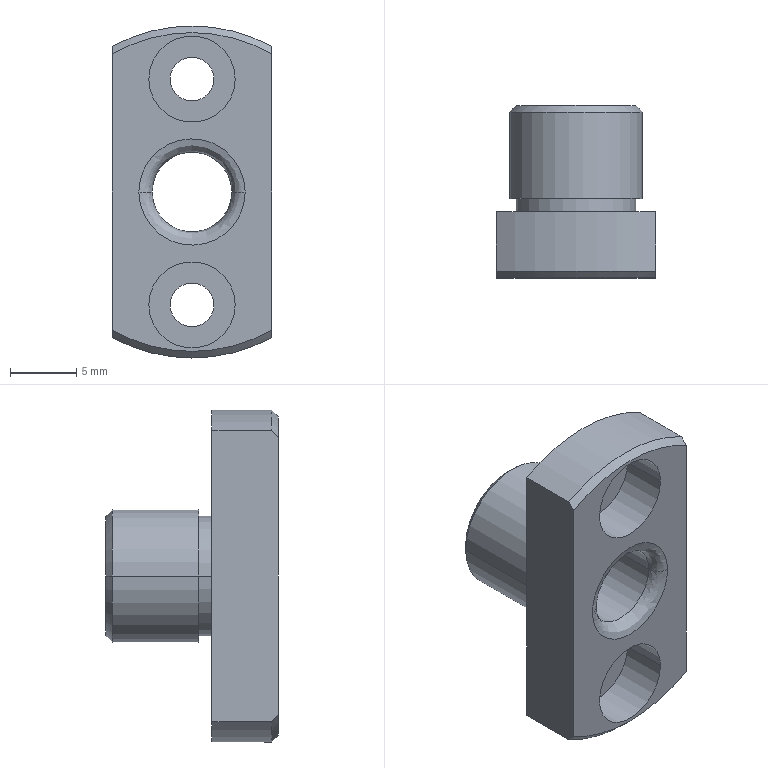Component | SolidWorks | F-JBNF10-P6-L8-1 | 1 solid | 30 faces | box 12 x 13 x 25 mm | volume 1417 mm3 | cylinder 16 | plane 8 | cone 4 | spline 2 | commonest cylinder face diameters 6.5 x4 3.3 x4 6 x2 10 x2 9 x2 25 x2
STEP:
#1=COLOUR_RGB('',0.7922,0.8196,0.9333);
#2=FILL_AREA_STYLE_COLOUR('',#1);
#3=FILL_AREA_STYLE('',(#2));
#4=SURFACE_STYLE_FILL_AREA(#3);
#5=SURFACE_SIDE_STYLE('',(#4));
#6=SURFACE_STYLE_USAGE(.BOTH.,#5);
#7=PRESENTATION_STYLE_ASSIGNMENT((#6));
#8=CARTESIAN_POINT('',(0.8391,-1.313,4.871));
#9=VERTEX_POINT('',#8);
#10=CARTESIAN_POINT('',(0.5241,-1.313,4.871));
#11=VERTEX_POINT('',#10);
#12=CARTESIAN_POINT('',(0.8391,-1.313,4.871));
#13=CARTESIAN_POINT('',(0.8391,-1.313,5.186));
#14=CARTESIAN_POINT('',(0.5241,-1.313,5.186));
#15=CARTESIAN_POINT('',(0.5241,-1.313,4.871));
#16=(BOUNDED_CURVE()B_SPLINE_CURVE(3,(#12,#13,#14,#15),.UNSPECIFIED.,.F.,.F.)B_SPLINE_CURVE_WITH_KNOTS((4,4),(0.,0.5),.UNSPECIFIED.)CURVE()GEOMETRIC_REPRESENTATION_ITEM()RATIONAL_B_SPLINE_CURVE((1.,0.3333,0.3333,1.))REPRESENTATION_ITEM(''));
#17=EDGE_CURVE('',#9,#11,#16,.T.);
#18=ORIENTED_EDGE('',*,*,#17,.T.);
#19=CARTESIAN_POINT('',(0.5635,-1.273,4.871));
#20=VERTEX_POINT('',#19);
#21=CARTESIAN_POINT('',(0.5241,-1.273,4.871));
#22=DIRECTION('',(-0.,0.,1.));
#23=DIRECTION('',(-1.,0.,0.));
#24=AXIS2_PLACEMENT_3D('',#21,#22,#23);
#25=CIRCLE('',#24,0.03937);
#26=EDGE_CURVE('',#11,#20,#25,.T.);
#27=ORIENTED_EDGE('',*,*,#26,.T.);
#28=CARTESIAN_POINT('',(0.7997,-1.273,4.871));
#29=VERTEX_POINT('',#28);
#30=CARTESIAN_POINT('',(0.6816,-1.273,4.871));
#31=DIRECTION('',(0.,1.,0.));
#32=DIRECTION('',(-1.,0.,0.));
#33=AXIS2_PLACEMENT_3D('',#30,#31,#32);
#34=CIRCLE('',#33,0.1181);
#35=EDGE_CURVE('',#20,#29,#34,.T.);
#36=ORIENTED_EDGE('',*,*,#35,.T.);
#37=CARTESIAN_POINT('',(0.8391,-1.273,4.871));
#38=DIRECTION('',(0.,0.,-1.));
#39=DIRECTION('',(1.,0.,0.));
#40=AXIS2_PLACEMENT_3D('',#37,#38,#39);
#41=CIRCLE('',#40,0.03937);
#42=EDGE_CURVE('',#9,#29,#41,.T.);
#43=ORIENTED_EDGE('',*,*,#42,.F.);
#44=EDGE_LOOP('',(#18,#27,#36,#43));
#45=FACE_OUTER_BOUND('',#44,.T.);
#46=CARTESIAN_POINT('',(0.5241,-1.313,4.871));
#47=CARTESIAN_POINT('',(0.5241,-1.313,5.186));
#48=CARTESIAN_POINT('',(0.8391,-1.313,5.186));
#49=CARTESIAN_POINT('',(0.8391,-1.313,4.871));
#50=CARTESIAN_POINT('',(0.5472,-1.313,4.871));
#51=CARTESIAN_POINT('',(0.5472,-1.313,5.14));
#52=CARTESIAN_POINT('',(0.816,-1.313,5.14));
#53=CARTESIAN_POINT('',(0.816,-1.313,4.871));
#54=CARTESIAN_POINT('',(0.5635,-1.296,4.871));
#55=CARTESIAN_POINT('',(0.5635,-1.296,5.107));
#56=CARTESIAN_POINT('',(0.7997,-1.296,5.107));
#57=CARTESIAN_POINT('',(0.7997,-1.296,4.871));
#58=CARTESIAN_POINT('',(0.5635,-1.273,4.871));
#59=CARTESIAN_POINT('',(0.5635,-1.273,5.107));
#60=CARTESIAN_POINT('',(0.7997,-1.273,5.107));
#61=CARTESIAN_POINT('',(0.7997,-1.273,4.871));
#62=(BOUNDED_SURFACE()B_SPLINE_SURFACE(3,3,((#46,#47,#48,#49),(#50,#51,#52,#53),(#54,#55,#56,#57),(#58,#59,#60,#61)),.UNSPECIFIED.,.F.,.F.,.F.)B_SPLINE_SURFACE_WITH_KNOTS((4,4),(4,4),(0.,1.),(0.,1.),.UNSPECIFIED.)GEOMETRIC_REPRESENTATION_ITEM()RATIONAL_B_SPLINE_SURFACE(((1.,0.3333,0.3333,1.),(0.8047,0.2682,0.2682,0.8047),(0.8047,0.2682,0.2682,0.8047),(1.,0.3333,0.3333,1.)))REPRESENTATION_ITEM('')SURFACE());
#63=ADVANCED_FACE('',(#45),#62,.T.);
#64=CARTESIAN_POINT('',(0.7997,-0.8009,4.871));
#65=VERTEX_POINT('',#64);
#66=CARTESIAN_POINT('',(0.5635,-0.8009,4.871));
#67=VERTEX_POINT('',#66);
#68=CARTESIAN_POINT('',(0.6816,-0.8009,4.871));
#69=DIRECTION('',(0.,-1.,0.));
#70=DIRECTION('',(-1.,0.,0.));
#71=AXIS2_PLACEMENT_3D('',#68,#69,#70);
#72=CIRCLE('',#71,0.1181);
#73=EDGE_CURVE('',#65,#67,#72,.T.);
#74=ORIENTED_EDGE('',*,*,#73,.F.);
#75=CARTESIAN_POINT('',(0.7997,-0.8009,4.871));
#76=DIRECTION('',(0.,-1.,0.));
#77=VECTOR('',#76,39.37);
#78=LINE('',#75,#77);
#79=EDGE_CURVE('',#65,#29,#78,.T.);
#80=ORIENTED_EDGE('',*,*,#79,.T.);
#81=ORIENTED_EDGE('',*,*,#35,.F.);
#82=CARTESIAN_POINT('',(0.5635,-0.8009,4.871));
#83=DIRECTION('',(0.,-1.,0.));
#84=VECTOR('',#83,39.37);
#85=LINE('',#82,#84);
#86=EDGE_CURVE('',#67,#20,#85,.T.);
#87=ORIENTED_EDGE('',*,*,#86,.F.);
#88=EDGE_LOOP('',(#74,#80,#81,#87));
#89=FACE_OUTER_BOUND('',#88,.T.);
#90=CARTESIAN_POINT('',(0.6816,-0.8009,4.871));
#91=DIRECTION('',(0.,-1.,0.));
#92=DIRECTION('',(-1.,0.,0.));
#93=AXIS2_PLACEMENT_3D('',#90,#91,#92);
#94=CYLINDRICAL_SURFACE('',#93,0.1181);
#95=ADVANCED_FACE('',(#89),#94,.F.);
#96=CARTESIAN_POINT('',(0.8587,-0.8009,4.871));
#97=VERTEX_POINT('',#96);
#98=CARTESIAN_POINT('',(0.5044,-0.8009,4.871));
#99=VERTEX_POINT('',#98);
#100=CARTESIAN_POINT('',(0.6816,-0.8009,4.871));
#101=DIRECTION('',(0.,1.,0.));
#102=DIRECTION('',(-1.,0.,0.));
#103=AXIS2_PLACEMENT_3D('',#100,#101,#102);
#104=CIRCLE('',#103,0.1772);
#105=EDGE_CURVE('',#97,#99,#104,.T.);
#106=ORIENTED_EDGE('',*,*,#105,.F.);
#107=CARTESIAN_POINT('',(0.8784,-0.8206,4.871));
#108=VERTEX_POINT('',#107);
#109=CARTESIAN_POINT('',(0.8784,-0.8206,4.871));
#110=DIRECTION('',(0.7071,-0.7071,-0.));
#111=VECTOR('',#110,39.37);
#112=LINE('',#109,#111);
#113=EDGE_CURVE('',#97,#108,#112,.T.);
#114=ORIENTED_EDGE('',*,*,#113,.T.);
#115=CARTESIAN_POINT('',(0.4847,-0.8206,4.871));
#116=VERTEX_POINT('',#115);
#117=CARTESIAN_POINT('',(0.6816,-0.8206,4.871));
#118=DIRECTION('',(0.,1.,0.));
#119=DIRECTION('',(-1.,0.,0.));
#120=AXIS2_PLACEMENT_3D('',#117,#118,#119);
#121=CIRCLE('',#120,0.1969);
#122=EDGE_CURVE('',#108,#116,#121,.T.);
#123=ORIENTED_EDGE('',*,*,#122,.T.);
#124=CARTESIAN_POINT('',(0.4847,-0.8206,4.871));
#125=DIRECTION('',(-0.7071,-0.7071,0.));
#126=VECTOR('',#125,39.37);
#127=LINE('',#124,#126);
#128=EDGE_CURVE('',#99,#116,#127,.T.);
#129=ORIENTED_EDGE('',*,*,#128,.F.);
#130=EDGE_LOOP('',(#106,#114,#123,#129));
#131=FACE_OUTER_BOUND('',#130,.T.);
#132=CARTESIAN_POINT('',(0.6816,-0.8206,4.871));
#133=DIRECTION('',(0.,-1.,0.));
#134=DIRECTION('',(-1.,0.,0.));
#135=AXIS2_PLACEMENT_3D('',#132,#133,#134);
#136=CONICAL_SURFACE('',#135,0.1969,0.7854);
#137=ADVANCED_FACE('',(#131),#136,.T.);
#138=CARTESIAN_POINT('',(0.5536,-1.313,5.206));
#139=VERTEX_POINT('',#138);
#140=CARTESIAN_POINT('',(0.8095,-1.313,5.206));
#141=VERTEX_POINT('',#140);
#142=CARTESIAN_POINT('',(0.6816,-1.313,5.206));
#143=DIRECTION('',(0.,1.,0.));
#144=DIRECTION('',(1.,0.,0.));
#145=AXIS2_PLACEMENT_3D('',#142,#143,#144);
#146=CIRCLE('',#145,0.128);
#147=EDGE_CURVE('',#139,#141,#146,.T.);
#148=ORIENTED_EDGE('',*,*,#147,.F.);
#149=CARTESIAN_POINT('',(0.5536,-1.175,5.206));
#150=VERTEX_POINT('',#149);
#151=CARTESIAN_POINT('',(0.5536,-1.313,5.206));
#152=DIRECTION('',(0.,1.,0.));
#153=VECTOR('',#152,39.37);
#154=LINE('',#151,#153);
#155=EDGE_CURVE('',#139,#150,#154,.T.);
#156=ORIENTED_EDGE('',*,*,#155,.T.);
#157=CARTESIAN_POINT('',(0.8095,-1.175,5.206));
#158=VERTEX_POINT('',#157);
#159=CARTESIAN_POINT('',(0.6816,-1.175,5.206));
#160=DIRECTION('',(0.,-1.,0.));
#161=DIRECTION('',(1.,0.,0.));
#162=AXIS2_PLACEMENT_3D('',#159,#160,#161);
#163=CIRCLE('',#162,0.128);
#164=EDGE_CURVE('',#158,#150,#163,.T.);
#165=ORIENTED_EDGE('',*,*,#164,.F.);
#166=CARTESIAN_POINT('',(0.8095,-1.313,5.206));
#167=DIRECTION('',(0.,1.,0.));
#168=VECTOR('',#167,39.37);
#169=LINE('',#166,#168);
#170=EDGE_CURVE('',#141,#158,#169,.T.);
#171=ORIENTED_EDGE('',*,*,#170,.F.);
#172=EDGE_LOOP('',(#148,#156,#165,#171));
#173=FACE_OUTER_BOUND('',#172,.T.);
#174=CARTESIAN_POINT('',(0.6816,-1.313,5.206));
#175=DIRECTION('',(0.,1.,0.));
#176=DIRECTION('',(1.,0.,0.));
#177=AXIS2_PLACEMENT_3D('',#174,#175,#176);
#178=CYLINDRICAL_SURFACE('',#177,0.128);
#179=ADVANCED_FACE('',(#173),#178,.F.);
#180=CARTESIAN_POINT('',(0.8095,-1.175,4.536));
#181=VERTEX_POINT('',#180);
#182=CARTESIAN_POINT('',(0.5536,-1.175,4.536));
#183=VERTEX_POINT('',#182);
#184=CARTESIAN_POINT('',(0.6816,-1.175,4.536));
#185=DIRECTION('',(0.,-1.,0.));
#186=DIRECTION('',(-1.,0.,0.));
#187=AXIS2_PLACEMENT_3D('',#184,#185,#186);
#188=CIRCLE('',#187,0.128);
#189=EDGE_CURVE('',#181,#183,#188,.T.);
#190=ORIENTED_EDGE('',*,*,#189,.F.);
#191=CARTESIAN_POINT('',(0.8095,-1.313,4.536));
#192=VERTEX_POINT('',#191);
#193=CARTESIAN_POINT('',(0.8095,-1.116,4.536));
#194=DIRECTION('',(0.,-1.,0.));
#195=VECTOR('',#194,39.37);
#196=LINE('',#193,#195);
#197=EDGE_CURVE('',#181,#192,#196,.T.);
#198=ORIENTED_EDGE('',*,*,#197,.T.);
#199=CARTESIAN_POINT('',(0.5536,-1.313,4.536));
#200=VERTEX_POINT('',#199);
#201=CARTESIAN_POINT('',(0.6816,-1.313,4.536));
#202=DIRECTION('',(0.,1.,0.));
#203=DIRECTION('',(-1.,0.,0.));
#204=AXIS2_PLACEMENT_3D('',#201,#202,#203);
#205=CIRCLE('',#204,0.128);
#206=EDGE_CURVE('',#200,#192,#205,.T.);
#207=ORIENTED_EDGE('',*,*,#206,.F.);
#208=CARTESIAN_POINT('',(0.5536,-1.116,4.536));
#209=DIRECTION('',(0.,-1.,0.));
#210=VECTOR('',#209,39.37);
#211=LINE('',#208,#210);
#212=EDGE_CURVE('',#183,#200,#211,.T.);
#213=ORIENTED_EDGE('',*,*,#212,.F.);
#214=EDGE_LOOP('',(#190,#198,#207,#213));
#215=FACE_OUTER_BOUND('',#214,.T.);
#216=CARTESIAN_POINT('',(0.6816,-1.116,4.536));
#217=DIRECTION('',(0.,-1.,0.));
#218=DIRECTION('',(-1.,0.,0.));
#219=AXIS2_PLACEMENT_3D('',#216,#217,#218);
#220=CYLINDRICAL_SURFACE('',#219,0.128);
#221=ADVANCED_FACE('',(#215),#220,.F.);
#222=ORIENTED_EDGE('',*,*,#122,.F.);
#223=CARTESIAN_POINT('',(0.8784,-1.076,4.871));
#224=VERTEX_POINT('',#223);
#225=CARTESIAN_POINT('',(0.8784,-0.8009,4.871));
#226=DIRECTION('',(0.,-1.,0.));
#227=VECTOR('',#226,39.37);
#228=LINE('',#225,#227);
#229=EDGE_CURVE('',#108,#224,#228,.T.);
#230=ORIENTED_EDGE('',*,*,#229,.T.);
#231=CARTESIAN_POINT('',(0.4847,-1.076,4.871));
#232=VERTEX_POINT('',#231);
#233=CARTESIAN_POINT('',(0.6816,-1.076,4.871));
#234=DIRECTION('',(0.,1.,0.));
#235=DIRECTION('',(-1.,0.,0.));
#236=AXIS2_PLACEMENT_3D('',#233,#234,#235);
#237=CIRCLE('',#236,0.1969);
#238=EDGE_CURVE('',#224,#232,#237,.T.);
#239=ORIENTED_EDGE('',*,*,#238,.T.);
#240=CARTESIAN_POINT('',(0.4847,-0.8009,4.871));
#241=DIRECTION('',(0.,-1.,0.));
#242=VECTOR('',#241,39.37);
#243=LINE('',#240,#242);
#244=EDGE_CURVE('',#116,#232,#243,.T.);
#245=ORIENTED_EDGE('',*,*,#244,.F.);
#246=EDGE_LOOP('',(#222,#230,#239,#245));
#247=FACE_OUTER_BOUND('',#246,.T.);
#248=CARTESIAN_POINT('',(0.6816,-0.8009,4.871));
#249=DIRECTION('',(0.,-1.,0.));
#250=DIRECTION('',(-1.,0.,0.));
#251=AXIS2_PLACEMENT_3D('',#248,#249,#250);
#252=CYLINDRICAL_SURFACE('',#251,0.1969);
#253=ADVANCED_FACE('',(#247),#252,.T.);
#254=CARTESIAN_POINT('',(0.6166,-1.175,5.206));
#255=VERTEX_POINT('',#254);
#256=CARTESIAN_POINT('',(0.7465,-1.175,5.206));
#257=VERTEX_POINT('',#256);
#258=CARTESIAN_POINT('',(0.6816,-1.175,5.206));
#259=DIRECTION('',(0.,1.,0.));
#260=DIRECTION('',(1.,0.,0.));
#261=AXIS2_PLACEMENT_3D('',#258,#259,#260);
#262=CIRCLE('',#261,0.06496);
#263=EDGE_CURVE('',#255,#257,#262,.T.);
#264=ORIENTED_EDGE('',*,*,#263,.F.);
#265=CARTESIAN_POINT('',(0.6166,-1.116,5.206));
#266=VERTEX_POINT('',#265);
#267=CARTESIAN_POINT('',(0.6166,-1.313,5.206));
#268=DIRECTION('',(0.,1.,0.));
#269=VECTOR('',#268,39.37);
#270=LINE('',#267,#269);
#271=EDGE_CURVE('',#255,#266,#270,.T.);
#272=ORIENTED_EDGE('',*,*,#271,.T.);
#273=CARTESIAN_POINT('',(0.7465,-1.116,5.206));
#274=VERTEX_POINT('',#273);
#275=CARTESIAN_POINT('',(0.6816,-1.116,5.206));
#276=DIRECTION('',(0.,-1.,0.));
#277=DIRECTION('',(1.,0.,0.));
#278=AXIS2_PLACEMENT_3D('',#275,#276,#277);
#279=CIRCLE('',#278,0.06496);
#280=EDGE_CURVE('',#274,#266,#279,.T.);
#281=ORIENTED_EDGE('',*,*,#280,.F.);
#282=CARTESIAN_POINT('',(0.7465,-1.313,5.206));
#283=DIRECTION('',(0.,1.,0.));
#284=VECTOR('',#283,39.37);
#285=LINE('',#282,#284);
#286=EDGE_CURVE('',#257,#274,#285,.T.);
#287=ORIENTED_EDGE('',*,*,#286,.F.);
#288=EDGE_LOOP('',(#264,#272,#281,#287));
#289=FACE_OUTER_BOUND('',#288,.T.);
#290=CARTESIAN_POINT('',(0.6816,-1.313,5.206));
#291=DIRECTION('',(0.,1.,0.));
#292=DIRECTION('',(1.,0.,0.));
#293=AXIS2_PLACEMENT_3D('',#290,#291,#292);
#294=CYLINDRICAL_SURFACE('',#293,0.06496);
#295=ADVANCED_FACE('',(#289),#294,.F.);
#296=CARTESIAN_POINT('',(0.8587,-1.076,4.871));
#297=VERTEX_POINT('',#296);
#298=CARTESIAN_POINT('',(0.5044,-1.076,4.871));
#299=VERTEX_POINT('',#298);
#300=CARTESIAN_POINT('',(0.6816,-1.076,4.871));
#301=DIRECTION('',(0.,1.,0.));
#302=DIRECTION('',(-1.,0.,0.));
#303=AXIS2_PLACEMENT_3D('',#300,#301,#302);
#304=CIRCLE('',#303,0.1772);
#305=EDGE_CURVE('',#297,#299,#304,.T.);
#306=ORIENTED_EDGE('',*,*,#305,.F.);
#307=CARTESIAN_POINT('',(0.8587,-1.116,4.871));
#308=VERTEX_POINT('',#307);
#309=CARTESIAN_POINT('',(0.8587,-0.8009,4.871));
#310=DIRECTION('',(0.,-1.,0.));
#311=VECTOR('',#310,39.37);
#312=LINE('',#309,#311);
#313=EDGE_CURVE('',#297,#308,#312,.T.);
#314=ORIENTED_EDGE('',*,*,#313,.T.);
#315=CARTESIAN_POINT('',(0.5044,-1.116,4.871));
#316=VERTEX_POINT('',#315);
#317=CARTESIAN_POINT('',(0.6816,-1.116,4.871));
#318=DIRECTION('',(0.,-1.,0.));
#319=DIRECTION('',(-1.,0.,0.));
#320=AXIS2_PLACEMENT_3D('',#317,#318,#319);
#321=CIRCLE('',#320,0.1772);
#322=EDGE_CURVE('',#316,#308,#321,.T.);
#323=ORIENTED_EDGE('',*,*,#322,.F.);
#324=CARTESIAN_POINT('',(0.5044,-0.8009,4.871));
#325=DIRECTION('',(0.,-1.,0.));
#326=VECTOR('',#325,39.37);
#327=LINE('',#324,#326);
#328=EDGE_CURVE('',#299,#316,#327,.T.);
#329=ORIENTED_EDGE('',*,*,#328,.F.);
#330=EDGE_LOOP('',(#306,#314,#323,#329));
#331=FACE_OUTER_BOUND('',#330,.T.);
#332=CARTESIAN_POINT('',(0.6816,-0.8009,4.871));
#333=DIRECTION('',(0.,-1.,0.));
#334=DIRECTION('',(-1.,0.,0.));
#335=AXIS2_PLACEMENT_3D('',#332,#333,#334);
#336=CYLINDRICAL_SURFACE('',#335,0.1772);
#337=ADVANCED_FACE('',(#331),#336,.T.);
#338=CARTESIAN_POINT('',(0.7465,-1.116,4.536));
#339=VERTEX_POINT('',#338);
#340=CARTESIAN_POINT('',(0.6166,-1.116,4.536));
#341=VERTEX_POINT('',#340);
#342=CARTESIAN_POINT('',(0.6816,-1.116,4.536));
#343=DIRECTION('',(0.,-1.,0.));
#344=DIRECTION('',(-1.,0.,0.));
#345=AXIS2_PLACEMENT_3D('',#342,#343,#344);
#346=CIRCLE('',#345,0.06496);
#347=EDGE_CURVE('',#339,#341,#346,.T.);
#348=ORIENTED_EDGE('',*,*,#347,.F.);
#349=CARTESIAN_POINT('',(0.7465,-1.175,4.536));
#350=VERTEX_POINT('',#349);
#351=CARTESIAN_POINT('',(0.7465,-1.116,4.536));
#352=DIRECTION('',(0.,-1.,0.));
#353=VECTOR('',#352,39.37);
#354=LINE('',#351,#353);
#355=EDGE_CURVE('',#339,#350,#354,.T.);
#356=ORIENTED_EDGE('',*,*,#355,.T.);
#357=CARTESIAN_POINT('',(0.6166,-1.175,4.536));
#358=VERTEX_POINT('',#357);
#359=CARTESIAN_POINT('',(0.6816,-1.175,4.536));
#360=DIRECTION('',(0.,1.,0.));
#361=DIRECTION('',(-1.,0.,0.));
#362=AXIS2_PLACEMENT_3D('',#359,#360,#361);
#363=CIRCLE('',#362,0.06496);
#364=EDGE_CURVE('',#358,#350,#363,.T.);
#365=ORIENTED_EDGE('',*,*,#364,.F.);
#366=CARTESIAN_POINT('',(0.6166,-1.116,4.536));
#367=DIRECTION('',(0.,-1.,0.));
#368=VECTOR('',#367,39.37);
#369=LINE('',#366,#368);
#370=EDGE_CURVE('',#341,#358,#369,.T.);
#371=ORIENTED_EDGE('',*,*,#370,.F.);
#372=EDGE_LOOP('',(#348,#356,#365,#371));
#373=FACE_OUTER_BOUND('',#372,.T.);
#374=CARTESIAN_POINT('',(0.6816,-1.116,4.536));
#375=DIRECTION('',(0.,-1.,0.));
#376=DIRECTION('',(-1.,0.,0.));
#377=AXIS2_PLACEMENT_3D('',#374,#375,#376);
#378=CYLINDRICAL_SURFACE('',#377,0.06496);
#379=ADVANCED_FACE('',(#373),#378,.F.);
#380=ORIENTED_EDGE('',*,*,#79,.F.);
#381=CARTESIAN_POINT('',(0.6816,-0.8009,4.871));
#382=DIRECTION('',(0.,-1.,0.));
#383=DIRECTION('',(-1.,0.,0.));
#384=AXIS2_PLACEMENT_3D('',#381,#382,#383);
#385=CIRCLE('',#384,0.1181);
#386=EDGE_CURVE('',#67,#65,#385,.T.);
#387=ORIENTED_EDGE('',*,*,#386,.F.);
#388=ORIENTED_EDGE('',*,*,#86,.T.);
#389=CARTESIAN_POINT('',(0.6816,-1.273,4.871));
#390=DIRECTION('',(0.,1.,0.));
#391=DIRECTION('',(-1.,0.,0.));
#392=AXIS2_PLACEMENT_3D('',#389,#390,#391);
#393=CIRCLE('',#392,0.1181);
#394=EDGE_CURVE('',#29,#20,#393,.T.);
#395=ORIENTED_EDGE('',*,*,#394,.F.);
#396=EDGE_LOOP('',(#380,#387,#388,#395));
#397=FACE_OUTER_BOUND('',#396,.T.);
#398=CARTESIAN_POINT('',(0.6816,-0.8009,4.871));
#399=DIRECTION('',(0.,-1.,0.));
#400=DIRECTION('',(-1.,0.,0.));
#401=AXIS2_PLACEMENT_3D('',#398,#399,#400);
#402=CYLINDRICAL_SURFACE('',#401,0.1181);
#403=ADVANCED_FACE('',(#397),#402,.F.);
#404=ORIENTED_EDGE('',*,*,#26,.F.);
#405=CARTESIAN_POINT('',(0.5241,-1.313,4.871));
#406=CARTESIAN_POINT('',(0.5241,-1.313,4.556));
#407=CARTESIAN_POINT('',(0.8391,-1.313,4.556));
#408=CARTESIAN_POINT('',(0.8391,-1.313,4.871));
#409=(BOUNDED_CURVE()B_SPLINE_CURVE(3,(#405,#406,#407,#408),.UNSPECIFIED.,.F.,.F.)B_SPLINE_CURVE_WITH_KNOTS((4,4),(0.5,1.),.UNSPECIFIED.)CURVE()GEOMETRIC_REPRESENTATION_ITEM()RATIONAL_B_SPLINE_CURVE((1.,0.3333,0.3333,1.))REPRESENTATION_ITEM(''));
#410=EDGE_CURVE('',#11,#9,#409,.T.);
#411=ORIENTED_EDGE('',*,*,#410,.T.);
#412=ORIENTED_EDGE('',*,*,#42,.T.);
#413=ORIENTED_EDGE('',*,*,#394,.T.);
#414=EDGE_LOOP('',(#404,#411,#412,#413));
#415=FACE_OUTER_BOUND('',#414,.T.);
#416=CARTESIAN_POINT('',(0.8391,-1.313,4.871));
#417=CARTESIAN_POINT('',(0.8391,-1.313,4.556));
#418=CARTESIAN_POINT('',(0.5241,-1.313,4.556));
#419=CARTESIAN_POINT('',(0.5241,-1.313,4.871));
#420=CARTESIAN_POINT('',(0.816,-1.313,4.871));
#421=CARTESIAN_POINT('',(0.816,-1.313,4.602));
#422=CARTESIAN_POINT('',(0.5472,-1.313,4.602));
#423=CARTESIAN_POINT('',(0.5472,-1.313,4.871));
#424=CARTESIAN_POINT('',(0.7997,-1.296,4.871));
#425=CARTESIAN_POINT('',(0.7997,-1.296,4.635));
#426=CARTESIAN_POINT('',(0.5635,-1.296,4.635));
#427=CARTESIAN_POINT('',(0.5635,-1.296,4.871));
#428=CARTESIAN_POINT('',(0.7997,-1.273,4.871));
#429=CARTESIAN_POINT('',(0.7997,-1.273,4.635));
#430=CARTESIAN_POINT('',(0.5635,-1.273,4.635));
#431=CARTESIAN_POINT('',(0.5635,-1.273,4.871));
#432=(BOUNDED_SURFACE()B_SPLINE_SURFACE(3,3,((#416,#417,#418,#419),(#420,#421,#422,#423),(#424,#425,#426,#427),(#428,#429,#430,#431)),.UNSPECIFIED.,.F.,.F.,.F.)B_SPLINE_SURFACE_WITH_KNOTS((4,4),(4,4),(0.,1.),(0.,1.),.UNSPECIFIED.)GEOMETRIC_REPRESENTATION_ITEM()RATIONAL_B_SPLINE_SURFACE(((1.,0.3333,0.3333,1.),(0.8047,0.2682,0.2682,0.8047),(0.8047,0.2682,0.2682,0.8047),(1.,0.3333,0.3333,1.)))REPRESENTATION_ITEM('')SURFACE());
#433=ADVANCED_FACE('',(#415),#432,.T.);
#434=ORIENTED_EDGE('',*,*,#386,.T.);
#435=ORIENTED_EDGE('',*,*,#73,.T.);
#436=EDGE_LOOP('',(#434,#435));
#437=FACE_BOUND('',#436,.T.);
#438=CARTESIAN_POINT('',(0.6816,-0.8009,4.871));
#439=DIRECTION('',(0.,1.,0.));
#440=DIRECTION('',(-1.,0.,0.));
#441=AXIS2_PLACEMENT_3D('',#438,#439,#440);
#442=CIRCLE('',#441,0.1772);
#443=EDGE_CURVE('',#99,#97,#442,.T.);
#444=ORIENTED_EDGE('',*,*,#443,.T.);
#445=ORIENTED_EDGE('',*,*,#105,.T.);
#446=EDGE_LOOP('',(#444,#445));
#447=FACE_OUTER_BOUND('',#446,.T.);
#448=CARTESIAN_POINT('',(0.6816,-0.8009,4.753));
#449=DIRECTION('',(0.,1.,0.));
#450=DIRECTION('',(1.,0.,0.));
#451=AXIS2_PLACEMENT_3D('',#448,#449,#450);
#452=PLANE('',#451);
#453=ADVANCED_FACE('',(#437,#447),#452,.T.);
#454=CARTESIAN_POINT('',(0.6816,-1.313,5.206));
#455=DIRECTION('',(0.,1.,0.));
#456=DIRECTION('',(1.,0.,0.));
#457=AXIS2_PLACEMENT_3D('',#454,#455,#456);
#458=CIRCLE('',#457,0.128);
#459=EDGE_CURVE('',#141,#139,#458,.T.);
#460=ORIENTED_EDGE('',*,*,#459,.T.);
#461=ORIENTED_EDGE('',*,*,#147,.T.);
#462=EDGE_LOOP('',(#460,#461));
#463=FACE_BOUND('',#462,.T.);
#464=CARTESIAN_POINT('',(0.9178,-1.313,5.28));
#465=VERTEX_POINT('',#464);
#466=CARTESIAN_POINT('',(0.4454,-1.313,5.28));
#467=VERTEX_POINT('',#466);
#468=CARTESIAN_POINT('',(0.6816,-1.313,4.871));
#469=DIRECTION('',(0.,-1.,0.));
#470=DIRECTION('',(1.,0.,-0.));
#471=AXIS2_PLACEMENT_3D('',#468,#469,#470);
#472=CIRCLE('',#471,0.4724);
#473=EDGE_CURVE('',#465,#467,#472,.T.);
#474=ORIENTED_EDGE('',*,*,#473,.T.);
#475=CARTESIAN_POINT('',(0.4454,-1.313,4.462));
#476=VERTEX_POINT('',#475);
#477=CARTESIAN_POINT('',(0.4454,-1.313,4.398));
#478=DIRECTION('',(0.,0.,-1.));
#479=VECTOR('',#478,39.37);
#480=LINE('',#477,#479);
#481=EDGE_CURVE('',#467,#476,#480,.T.);
#482=ORIENTED_EDGE('',*,*,#481,.T.);
#483=CARTESIAN_POINT('',(0.9178,-1.313,4.462));
#484=VERTEX_POINT('',#483);
#485=CARTESIAN_POINT('',(0.6816,-1.313,4.871));
#486=DIRECTION('',(0.,-1.,0.));
#487=DIRECTION('',(1.,0.,0.));
#488=AXIS2_PLACEMENT_3D('',#485,#486,#487);
#489=CIRCLE('',#488,0.4724);
#490=EDGE_CURVE('',#476,#484,#489,.T.);
#491=ORIENTED_EDGE('',*,*,#490,.T.);
#492=CARTESIAN_POINT('',(0.9178,-1.313,4.398));
#493=DIRECTION('',(0.,0.,1.));
#494=VECTOR('',#493,39.37);
#495=LINE('',#492,#494);
#496=EDGE_CURVE('',#484,#465,#495,.T.);
#497=ORIENTED_EDGE('',*,*,#496,.T.);
#498=EDGE_LOOP('',(#474,#482,#491,#497));
#499=FACE_OUTER_BOUND('',#498,.T.);
#500=ORIENTED_EDGE('',*,*,#206,.T.);
#501=CARTESIAN_POINT('',(0.6816,-1.313,4.536));
#502=DIRECTION('',(0.,1.,0.));
#503=DIRECTION('',(-1.,0.,0.));
#504=AXIS2_PLACEMENT_3D('',#501,#502,#503);
#505=CIRCLE('',#504,0.128);
#506=EDGE_CURVE('',#192,#200,#505,.T.);
#507=ORIENTED_EDGE('',*,*,#506,.T.);
#508=EDGE_LOOP('',(#500,#507));
#509=FACE_BOUND('',#508,.T.);
#510=ORIENTED_EDGE('',*,*,#17,.F.);
#511=ORIENTED_EDGE('',*,*,#410,.F.);
#512=EDGE_LOOP('',(#510,#511));
#513=FACE_BOUND('',#512,.T.);
#514=CARTESIAN_POINT('',(0.6816,-1.313,4.398));
#515=DIRECTION('',(0.,-1.,0.));
#516=DIRECTION('',(-1.,0.,0.));
#517=AXIS2_PLACEMENT_3D('',#514,#515,#516);
#518=PLANE('',#517);
#519=ADVANCED_FACE('',(#463,#499,#509,#513),#518,.T.);
#520=ORIENTED_EDGE('',*,*,#113,.F.);
#521=ORIENTED_EDGE('',*,*,#443,.F.);
#522=ORIENTED_EDGE('',*,*,#128,.T.);
#523=CARTESIAN_POINT('',(0.6816,-0.8206,4.871));
#524=DIRECTION('',(0.,1.,0.));
#525=DIRECTION('',(-1.,0.,0.));
#526=AXIS2_PLACEMENT_3D('',#523,#524,#525);
#527=CIRCLE('',#526,0.1969);
#528=EDGE_CURVE('',#116,#108,#527,.T.);
#529=ORIENTED_EDGE('',*,*,#528,.T.);
#530=EDGE_LOOP('',(#520,#521,#522,#529));
#531=FACE_OUTER_BOUND('',#530,.T.);
#532=CARTESIAN_POINT('',(0.6816,-0.8206,4.871));
#533=DIRECTION('',(0.,-1.,0.));
#534=DIRECTION('',(-1.,0.,0.));
#535=AXIS2_PLACEMENT_3D('',#532,#533,#534);
#536=CONICAL_SURFACE('',#535,0.1969,0.7854);
#537=ADVANCED_FACE('',(#531),#536,.T.);
#538=ORIENTED_EDGE('',*,*,#155,.F.);
#539=ORIENTED_EDGE('',*,*,#459,.F.);
#540=ORIENTED_EDGE('',*,*,#170,.T.);
#541=CARTESIAN_POINT('',(0.6816,-1.175,5.206));
#542=DIRECTION('',(0.,-1.,0.));
#543=DIRECTION('',(1.,0.,0.));
#544=AXIS2_PLACEMENT_3D('',#541,#542,#543);
#545=CIRCLE('',#544,0.128);
#546=EDGE_CURVE('',#150,#158,#545,.T.);
#547=ORIENTED_EDGE('',*,*,#546,.F.);
#548=EDGE_LOOP('',(#538,#539,#540,#547));
#549=FACE_OUTER_BOUND('',#548,.T.);
#550=CARTESIAN_POINT('',(0.6816,-1.313,5.206));
#551=DIRECTION('',(0.,1.,0.));
#552=DIRECTION('',(1.,0.,0.));
#553=AXIS2_PLACEMENT_3D('',#550,#551,#552);
#554=CYLINDRICAL_SURFACE('',#553,0.128);
#555=ADVANCED_FACE('',(#549),#554,.F.);
#556=CARTESIAN_POINT('',(0.4454,-1.293,4.439));
#557=VERTEX_POINT('',#556);
#558=CARTESIAN_POINT('',(0.4454,-1.313,4.462));
#559=CARTESIAN_POINT('',(0.4454,-1.306,4.454));
#560=CARTESIAN_POINT('',(0.4454,-1.3,4.447));
#561=CARTESIAN_POINT('',(0.4454,-1.293,4.439));
#562=B_SPLINE_CURVE_WITH_KNOTS('',3,(#558,#559,#560,#561),.UNSPECIFIED.,.F.,.F.,(4,4),(0.,0.0007609),.UNSPECIFIED.);
#563=EDGE_CURVE('',#476,#557,#562,.T.);
#564=ORIENTED_EDGE('',*,*,#563,.F.);
#565=ORIENTED_EDGE('',*,*,#481,.F.);
#566=CARTESIAN_POINT('',(0.4454,-1.293,5.303));
#567=VERTEX_POINT('',#566);
#568=CARTESIAN_POINT('',(0.4454,-1.293,5.303));
#569=CARTESIAN_POINT('',(0.4454,-1.3,5.295));
#570=CARTESIAN_POINT('',(0.4454,-1.306,5.288));
#571=CARTESIAN_POINT('',(0.4454,-1.313,5.28));
#572=B_SPLINE_CURVE_WITH_KNOTS('',3,(#568,#569,#570,#571),.UNSPECIFIED.,.F.,.F.,(4,4),(0.,0.0007609),.UNSPECIFIED.);
#573=EDGE_CURVE('',#567,#467,#572,.T.);
#574=ORIENTED_EDGE('',*,*,#573,.F.);
#575=CARTESIAN_POINT('',(0.4454,-1.116,5.303));
#576=VERTEX_POINT('',#575);
#577=CARTESIAN_POINT('',(0.4454,-1.116,5.303));
#578=DIRECTION('',(0.,-1.,0.));
#579=VECTOR('',#578,39.37);
#580=LINE('',#577,#579);
#581=EDGE_CURVE('',#576,#567,#580,.T.);
#582=ORIENTED_EDGE('',*,*,#581,.F.);
#583=CARTESIAN_POINT('',(0.4454,-1.116,4.439));
#584=VERTEX_POINT('',#583);
#585=CARTESIAN_POINT('',(0.4454,-1.116,4.379));
#586=DIRECTION('',(0.,0.,1.));
#587=VECTOR('',#586,39.37);
#588=LINE('',#585,#587);
#589=EDGE_CURVE('',#584,#576,#588,.T.);
#590=ORIENTED_EDGE('',*,*,#589,.F.);
#591=CARTESIAN_POINT('',(0.4454,-1.116,4.439));
#592=DIRECTION('',(0.,1.,0.));
#593=VECTOR('',#592,39.37);
#594=LINE('',#591,#593);
#595=EDGE_CURVE('',#557,#584,#594,.T.);
#596=ORIENTED_EDGE('',*,*,#595,.F.);
#597=EDGE_LOOP('',(#564,#565,#574,#582,#590,#596));
#598=FACE_OUTER_BOUND('',#597,.T.);
#599=CARTESIAN_POINT('',(0.4454,-1.116,4.379));
#600=DIRECTION('',(1.,0.,0.));
#601=DIRECTION('',(0.,-1.,0.));
#602=AXIS2_PLACEMENT_3D('',#599,#600,#601);
#603=PLANE('',#602);
#604=ADVANCED_FACE('',(#598),#603,.F.);
#605=CARTESIAN_POINT('',(0.9178,-1.293,5.303));
#606=VERTEX_POINT('',#605);
#607=CARTESIAN_POINT('',(0.9178,-1.313,5.28));
#608=CARTESIAN_POINT('',(0.9178,-1.306,5.288));
#609=CARTESIAN_POINT('',(0.9178,-1.3,5.295));
#610=CARTESIAN_POINT('',(0.9178,-1.293,5.303));
#611=B_SPLINE_CURVE_WITH_KNOTS('',3,(#607,#608,#609,#610),.UNSPECIFIED.,.F.,.F.,(4,4),(0.,0.0007609),.UNSPECIFIED.);
#612=EDGE_CURVE('',#465,#606,#611,.T.);
#613=ORIENTED_EDGE('',*,*,#612,.T.);
#614=CARTESIAN_POINT('',(0.6816,-1.293,4.871));
#615=DIRECTION('',(0.,-1.,0.));
#616=DIRECTION('',(1.,0.,-0.));
#617=AXIS2_PLACEMENT_3D('',#614,#615,#616);
#618=CIRCLE('',#617,0.4921);
#619=EDGE_CURVE('',#606,#567,#618,.T.);
#620=ORIENTED_EDGE('',*,*,#619,.T.);
#621=ORIENTED_EDGE('',*,*,#573,.T.);
#622=ORIENTED_EDGE('',*,*,#473,.F.);
#623=EDGE_LOOP('',(#613,#620,#621,#622));
#624=FACE_OUTER_BOUND('',#623,.T.);
#625=CARTESIAN_POINT('',(0.6816,-1.293,4.871));
#626=DIRECTION('',(0.,1.,0.));
#627=DIRECTION('',(1.,0.,0.));
#628=AXIS2_PLACEMENT_3D('',#625,#626,#627);
#629=CONICAL_SURFACE('',#628,0.4921,0.7854);
#630=ADVANCED_FACE('',(#624),#629,.T.);
#631=ORIENTED_EDGE('',*,*,#612,.F.);
#632=ORIENTED_EDGE('',*,*,#496,.F.);
#633=CARTESIAN_POINT('',(0.9178,-1.293,4.439));
#634=VERTEX_POINT('',#633);
#635=CARTESIAN_POINT('',(0.9178,-1.293,4.439));
#636=CARTESIAN_POINT('',(0.9178,-1.3,4.447));
#637=CARTESIAN_POINT('',(0.9178,-1.306,4.454));
#638=CARTESIAN_POINT('',(0.9178,-1.313,4.462));
#639=B_SPLINE_CURVE_WITH_KNOTS('',3,(#635,#636,#637,#638),.UNSPECIFIED.,.F.,.F.,(4,4),(0.,0.0007609),.UNSPECIFIED.);
#640=EDGE_CURVE('',#634,#484,#639,.T.);
#641=ORIENTED_EDGE('',*,*,#640,.F.);
#642=CARTESIAN_POINT('',(0.9178,-1.116,4.439));
#643=VERTEX_POINT('',#642);
#644=CARTESIAN_POINT('',(0.9178,-1.116,4.439));
#645=DIRECTION('',(0.,-1.,0.));
#646=VECTOR('',#645,39.37);
#647=LINE('',#644,#646);
#648=EDGE_CURVE('',#643,#634,#647,.T.);
#649=ORIENTED_EDGE('',*,*,#648,.F.);
#650=CARTESIAN_POINT('',(0.9178,-1.116,5.303));
#651=VERTEX_POINT('',#650);
#652=CARTESIAN_POINT('',(0.9178,-1.116,5.363));
#653=DIRECTION('',(0.,0.,-1.));
#654=VECTOR('',#653,39.37);
#655=LINE('',#652,#654);
#656=EDGE_CURVE('',#651,#643,#655,.T.);
#657=ORIENTED_EDGE('',*,*,#656,.F.);
#658=CARTESIAN_POINT('',(0.9178,-1.116,5.303));
#659=DIRECTION('',(0.,1.,0.));
#660=VECTOR('',#659,39.37);
#661=LINE('',#658,#660);
#662=EDGE_CURVE('',#606,#651,#661,.T.);
#663=ORIENTED_EDGE('',*,*,#662,.F.);
#664=EDGE_LOOP('',(#631,#632,#641,#649,#657,#663));
#665=FACE_OUTER_BOUND('',#664,.T.);
#666=CARTESIAN_POINT('',(0.9178,-1.116,5.363));
#667=DIRECTION('',(-1.,0.,0.));
#668=DIRECTION('',(0.,1.,0.));
#669=AXIS2_PLACEMENT_3D('',#666,#667,#668);
#670=PLANE('',#669);
#671=ADVANCED_FACE('',(#665),#670,.F.);
#672=ORIENTED_EDGE('',*,*,#563,.T.);
#673=CARTESIAN_POINT('',(0.6816,-1.293,4.871));
#674=DIRECTION('',(0.,-1.,0.));
#675=DIRECTION('',(1.,0.,0.));
#676=AXIS2_PLACEMENT_3D('',#673,#674,#675);
#677=CIRCLE('',#676,0.4921);
#678=EDGE_CURVE('',#557,#634,#677,.T.);
#679=ORIENTED_EDGE('',*,*,#678,.T.);
#680=ORIENTED_EDGE('',*,*,#640,.T.);
#681=ORIENTED_EDGE('',*,*,#490,.F.);
#682=EDGE_LOOP('',(#672,#679,#680,#681));
#683=FACE_OUTER_BOUND('',#682,.T.);
#684=CARTESIAN_POINT('',(0.6816,-1.293,4.871));
#685=DIRECTION('',(0.,1.,0.));
#686=DIRECTION('',(1.,0.,0.));
#687=AXIS2_PLACEMENT_3D('',#684,#685,#686);
#688=CONICAL_SURFACE('',#687,0.4921,0.7854);
#689=ADVANCED_FACE('',(#683),#688,.T.);
#690=ORIENTED_EDGE('',*,*,#197,.F.);
#691=CARTESIAN_POINT('',(0.6816,-1.175,4.536));
#692=DIRECTION('',(0.,-1.,0.));
#693=DIRECTION('',(-1.,0.,0.));
#694=AXIS2_PLACEMENT_3D('',#691,#692,#693);
#695=CIRCLE('',#694,0.128);
#696=EDGE_CURVE('',#183,#181,#695,.T.);
#697=ORIENTED_EDGE('',*,*,#696,.F.);
#698=ORIENTED_EDGE('',*,*,#212,.T.);
#699=ORIENTED_EDGE('',*,*,#506,.F.);
#700=EDGE_LOOP('',(#690,#697,#698,#699));
#701=FACE_OUTER_BOUND('',#700,.T.);
#702=CARTESIAN_POINT('',(0.6816,-1.116,4.536));
#703=DIRECTION('',(0.,-1.,0.));
#704=DIRECTION('',(-1.,0.,0.));
#705=AXIS2_PLACEMENT_3D('',#702,#703,#704);
#706=CYLINDRICAL_SURFACE('',#705,0.128);
#707=ADVANCED_FACE('',(#701),#706,.F.);
#708=ORIENTED_EDGE('',*,*,#229,.F.);
#709=ORIENTED_EDGE('',*,*,#528,.F.);
#710=ORIENTED_EDGE('',*,*,#244,.T.);
#711=CARTESIAN_POINT('',(0.6816,-1.076,4.871));
#712=DIRECTION('',(0.,1.,0.));
#713=DIRECTION('',(-1.,0.,0.));
#714=AXIS2_PLACEMENT_3D('',#711,#712,#713);
#715=CIRCLE('',#714,0.1969);
#716=EDGE_CURVE('',#232,#224,#715,.T.);
#717=ORIENTED_EDGE('',*,*,#716,.T.);
#718=EDGE_LOOP('',(#708,#709,#710,#717));
#719=FACE_OUTER_BOUND('',#718,.T.);
#720=CARTESIAN_POINT('',(0.6816,-0.8009,4.871));
#721=DIRECTION('',(0.,-1.,0.));
#722=DIRECTION('',(-1.,0.,0.));
#723=AXIS2_PLACEMENT_3D('',#720,#721,#722);
#724=CYLINDRICAL_SURFACE('',#723,0.1969);
#725=ADVANCED_FACE('',(#719),#724,.T.);
#726=CARTESIAN_POINT('',(0.6816,-1.175,5.206));
#727=DIRECTION('',(0.,1.,0.));
#728=DIRECTION('',(1.,0.,0.));
#729=AXIS2_PLACEMENT_3D('',#726,#727,#728);
#730=CIRCLE('',#729,0.06496);
#731=EDGE_CURVE('',#257,#255,#730,.T.);
#732=ORIENTED_EDGE('',*,*,#731,.T.);
#733=ORIENTED_EDGE('',*,*,#263,.T.);
#734=EDGE_LOOP('',(#732,#733));
#735=FACE_BOUND('',#734,.T.);
#736=ORIENTED_EDGE('',*,*,#164,.T.);
#737=ORIENTED_EDGE('',*,*,#546,.T.);
#738=EDGE_LOOP('',(#736,#737));
#739=FACE_OUTER_BOUND('',#738,.T.);
#740=CARTESIAN_POINT('',(0.6816,-1.175,5.27));
#741=DIRECTION('',(0.,-1.,0.));
#742=DIRECTION('',(-1.,0.,0.));
#743=AXIS2_PLACEMENT_3D('',#740,#741,#742);
#744=PLANE('',#743);
#745=ADVANCED_FACE('',(#735,#739),#744,.T.);
#746=ORIENTED_EDGE('',*,*,#595,.T.);
#747=CARTESIAN_POINT('',(0.6816,-1.116,4.871));
#748=DIRECTION('',(0.,-1.,0.));
#749=DIRECTION('',(-1.,0.,0.));
#750=AXIS2_PLACEMENT_3D('',#747,#748,#749);
#751=CIRCLE('',#750,0.4921);
#752=EDGE_CURVE('',#584,#643,#751,.T.);
#753=ORIENTED_EDGE('',*,*,#752,.T.);
#754=ORIENTED_EDGE('',*,*,#648,.T.);
#755=ORIENTED_EDGE('',*,*,#678,.F.);
#756=EDGE_LOOP('',(#746,#753,#754,#755));
#757=FACE_OUTER_BOUND('',#756,.T.);
#758=CARTESIAN_POINT('',(0.6816,-0.8009,4.871));
#759=DIRECTION('',(0.,-1.,0.));
#760=DIRECTION('',(-1.,0.,0.));
#761=AXIS2_PLACEMENT_3D('',#758,#759,#760);
#762=CYLINDRICAL_SURFACE('',#761,0.4921);
#763=ADVANCED_FACE('',(#757),#762,.T.);
#764=ORIENTED_EDGE('',*,*,#662,.T.);
#765=CARTESIAN_POINT('',(0.6816,-1.116,4.871));
#766=DIRECTION('',(0.,-1.,0.));
#767=DIRECTION('',(-1.,0.,0.));
#768=AXIS2_PLACEMENT_3D('',#765,#766,#767);
#769=CIRCLE('',#768,0.4921);
#770=EDGE_CURVE('',#651,#576,#769,.T.);
#771=ORIENTED_EDGE('',*,*,#770,.T.);
#772=ORIENTED_EDGE('',*,*,#581,.T.);
#773=ORIENTED_EDGE('',*,*,#619,.F.);
#774=EDGE_LOOP('',(#764,#771,#772,#773));
#775=FACE_OUTER_BOUND('',#774,.T.);
#776=CARTESIAN_POINT('',(0.6816,-0.8009,4.871));
#777=DIRECTION('',(0.,-1.,0.));
#778=DIRECTION('',(-1.,0.,0.));
#779=AXIS2_PLACEMENT_3D('',#776,#777,#778);
#780=CYLINDRICAL_SURFACE('',#779,0.4921);
#781=ADVANCED_FACE('',(#775),#780,.T.);
#782=ORIENTED_EDGE('',*,*,#280,.T.);
#783=CARTESIAN_POINT('',(0.6816,-1.116,5.206));
#784=DIRECTION('',(0.,-1.,0.));
#785=DIRECTION('',(1.,0.,0.));
#786=AXIS2_PLACEMENT_3D('',#783,#784,#785);
#787=CIRCLE('',#786,0.06496);
#788=EDGE_CURVE('',#266,#274,#787,.T.);
#789=ORIENTED_EDGE('',*,*,#788,.T.);
#790=EDGE_LOOP('',(#782,#789));
#791=FACE_BOUND('',#790,.T.);
#792=ORIENTED_EDGE('',*,*,#322,.T.);
#793=CARTESIAN_POINT('',(0.6816,-1.116,4.871));
#794=DIRECTION('',(0.,-1.,0.));
#795=DIRECTION('',(-1.,0.,0.));
#796=AXIS2_PLACEMENT_3D('',#793,#794,#795);
#797=CIRCLE('',#796,0.1772);
#798=EDGE_CURVE('',#308,#316,#797,.T.);
#799=ORIENTED_EDGE('',*,*,#798,.T.);
#800=EDGE_LOOP('',(#792,#799));
#801=FACE_BOUND('',#800,.T.);
#802=CARTESIAN_POINT('',(0.6816,-1.116,4.536));
#803=DIRECTION('',(0.,-1.,0.));
#804=DIRECTION('',(-1.,0.,0.));
#805=AXIS2_PLACEMENT_3D('',#802,#803,#804);
#806=CIRCLE('',#805,0.06496);
#807=EDGE_CURVE('',#341,#339,#806,.T.);
#808=ORIENTED_EDGE('',*,*,#807,.T.);
#809=ORIENTED_EDGE('',*,*,#347,.T.);
#810=EDGE_LOOP('',(#808,#809));
#811=FACE_BOUND('',#810,.T.);
#812=ORIENTED_EDGE('',*,*,#589,.T.);
#813=ORIENTED_EDGE('',*,*,#770,.F.);
#814=ORIENTED_EDGE('',*,*,#656,.T.);
#815=ORIENTED_EDGE('',*,*,#752,.F.);
#816=EDGE_LOOP('',(#812,#813,#814,#815));
#817=FACE_OUTER_BOUND('',#816,.T.);
#818=CARTESIAN_POINT('',(0.6816,-1.116,4.694));
#819=DIRECTION('',(0.,1.,0.));
#820=DIRECTION('',(1.,0.,0.));
#821=AXIS2_PLACEMENT_3D('',#818,#819,#820);
#822=PLANE('',#821);
#823=ADVANCED_FACE('',(#791,#801,#811,#817),#822,.T.);
#824=ORIENTED_EDGE('',*,*,#696,.T.);
#825=ORIENTED_EDGE('',*,*,#189,.T.);
#826=EDGE_LOOP('',(#824,#825));
#827=FACE_OUTER_BOUND('',#826,.T.);
#828=ORIENTED_EDGE('',*,*,#364,.T.);
#829=CARTESIAN_POINT('',(0.6816,-1.175,4.536));
#830=DIRECTION('',(0.,1.,0.));
#831=DIRECTION('',(-1.,0.,0.));
#832=AXIS2_PLACEMENT_3D('',#829,#830,#831);
#833=CIRCLE('',#832,0.06496);
#834=EDGE_CURVE('',#350,#358,#833,.T.);
#835=ORIENTED_EDGE('',*,*,#834,.T.);
#836=EDGE_LOOP('',(#828,#835));
#837=FACE_BOUND('',#836,.T.);
#838=CARTESIAN_POINT('',(0.6816,-1.175,4.408));
#839=DIRECTION('',(0.,-1.,0.));
#840=DIRECTION('',(-1.,0.,0.));
#841=AXIS2_PLACEMENT_3D('',#838,#839,#840);
#842=PLANE('',#841);
#843=ADVANCED_FACE('',(#827,#837),#842,.T.);
#844=ORIENTED_EDGE('',*,*,#716,.F.);
#845=ORIENTED_EDGE('',*,*,#238,.F.);
#846=EDGE_LOOP('',(#844,#845));
#847=FACE_OUTER_BOUND('',#846,.T.);
#848=CARTESIAN_POINT('',(0.6816,-1.076,4.871));
#849=DIRECTION('',(0.,1.,0.));
#850=DIRECTION('',(-1.,0.,0.));
#851=AXIS2_PLACEMENT_3D('',#848,#849,#850);
#852=CIRCLE('',#851,0.1772);
#853=EDGE_CURVE('',#299,#297,#852,.T.);
#854=ORIENTED_EDGE('',*,*,#853,.T.);
#855=ORIENTED_EDGE('',*,*,#305,.T.);
#856=EDGE_LOOP('',(#854,#855));
#857=FACE_BOUND('',#856,.T.);
#858=CARTESIAN_POINT('',(0.6816,-1.076,4.674));
#859=DIRECTION('',(0.,-1.,0.));
#860=DIRECTION('',(-1.,0.,0.));
#861=AXIS2_PLACEMENT_3D('',#858,#859,#860);
#862=PLANE('',#861);
#863=ADVANCED_FACE('',(#847,#857),#862,.T.);
#864=ORIENTED_EDGE('',*,*,#271,.F.);
#865=ORIENTED_EDGE('',*,*,#731,.F.);
#866=ORIENTED_EDGE('',*,*,#286,.T.);
#867=ORIENTED_EDGE('',*,*,#788,.F.);
#868=EDGE_LOOP('',(#864,#865,#866,#867));
#869=FACE_OUTER_BOUND('',#868,.T.);
#870=CARTESIAN_POINT('',(0.6816,-1.313,5.206));
#871=DIRECTION('',(0.,1.,0.));
#872=DIRECTION('',(1.,0.,0.));
#873=AXIS2_PLACEMENT_3D('',#870,#871,#872);
#874=CYLINDRICAL_SURFACE('',#873,0.06496);
#875=ADVANCED_FACE('',(#869),#874,.F.);
#876=ORIENTED_EDGE('',*,*,#313,.F.);
#877=ORIENTED_EDGE('',*,*,#853,.F.);
#878=ORIENTED_EDGE('',*,*,#328,.T.);
#879=ORIENTED_EDGE('',*,*,#798,.F.);
#880=EDGE_LOOP('',(#876,#877,#878,#879));
#881=FACE_OUTER_BOUND('',#880,.T.);
#882=CARTESIAN_POINT('',(0.6816,-0.8009,4.871));
#883=DIRECTION('',(0.,-1.,0.));
#884=DIRECTION('',(-1.,0.,0.));
#885=AXIS2_PLACEMENT_3D('',#882,#883,#884);
#886=CYLINDRICAL_SURFACE('',#885,0.1772);
#887=ADVANCED_FACE('',(#881),#886,.T.);
#888=ORIENTED_EDGE('',*,*,#355,.F.);
#889=ORIENTED_EDGE('',*,*,#807,.F.);
#890=ORIENTED_EDGE('',*,*,#370,.T.);
#891=ORIENTED_EDGE('',*,*,#834,.F.);
#892=EDGE_LOOP('',(#888,#889,#890,#891));
#893=FACE_OUTER_BOUND('',#892,.T.);
#894=CARTESIAN_POINT('',(0.6816,-1.116,4.536));
#895=DIRECTION('',(0.,-1.,0.));
#896=DIRECTION('',(-1.,0.,0.));
#897=AXIS2_PLACEMENT_3D('',#894,#895,#896);
#898=CYLINDRICAL_SURFACE('',#897,0.06496);
#899=ADVANCED_FACE('',(#893),#898,.F.);
#900=CLOSED_SHELL('',(#63,#95,#137,#179,#221,#253,#295,#337,#379,#403,#433,#453,#519,#537,#555,#604,#630,#671,#689,#707,#725,#745,#763,#781,#823,#843,#863,#875,#887,#899));
#901=MANIFOLD_SOLID_BREP('',#900);
#902=STYLED_ITEM('',(#7),#901);
#903=PRESENTATION_LAYER_ASSIGNMENT('','',(#902));
#904=(LENGTH_UNIT()NAMED_UNIT(*)SI_UNIT($,.METRE.));
#905=LENGTH_MEASURE_WITH_UNIT(LENGTH_MEASURE(0.0254),#904);
#906=DIMENSIONAL_EXPONENTS(1.,0.,0.,0.,0.,0.,0.);
#907=(CONVERSION_BASED_UNIT('',#905)LENGTH_UNIT()NAMED_UNIT(#906));
#908=UNCERTAINTY_MEASURE_WITH_UNIT(LENGTH_MEASURE(0.00001),#907,'','');
#909=(NAMED_UNIT(*)PLANE_ANGLE_UNIT()SI_UNIT($,.RADIAN.));
#910=(NAMED_UNIT(*)SI_UNIT($,.STERADIAN.)SOLID_ANGLE_UNIT());
#911=(GEOMETRIC_REPRESENTATION_CONTEXT(3)GLOBAL_UNCERTAINTY_ASSIGNED_CONTEXT((#908))GLOBAL_UNIT_ASSIGNED_CONTEXT((#907,#909,#910))REPRESENTATION_CONTEXT('',''));
#912=MECHANICAL_DESIGN_GEOMETRIC_PRESENTATION_REPRESENTATION('',(#902),#911);
#913=CARTESIAN_POINT('',(0.,0.,0.));
#914=DIRECTION('',(0.,0.,1.));
#915=DIRECTION('',(1.,0.,0.));
#916=AXIS2_PLACEMENT_3D('',#913,#914,#915);
#917=(LENGTH_UNIT()NAMED_UNIT(*)SI_UNIT($,.METRE.));
#918=LENGTH_MEASURE_WITH_UNIT(LENGTH_MEASURE(0.0254),#917);
#919=DIMENSIONAL_EXPONENTS(1.,0.,0.,0.,0.,0.,0.);
#920=(CONVERSION_BASED_UNIT('',#918)LENGTH_UNIT()NAMED_UNIT(#919));
#921=UNCERTAINTY_MEASURE_WITH_UNIT(LENGTH_MEASURE(0.00001),#920,'','');
#922=(NAMED_UNIT(*)PLANE_ANGLE_UNIT()SI_UNIT($,.RADIAN.));
#923=(NAMED_UNIT(*)SI_UNIT($,.STERADIAN.)SOLID_ANGLE_UNIT());
#924=(GEOMETRIC_REPRESENTATION_CONTEXT(3)GLOBAL_UNCERTAINTY_ASSIGNED_CONTEXT((#921))GLOBAL_UNIT_ASSIGNED_CONTEXT((#920,#922,#923))REPRESENTATION_CONTEXT('',''));
#925=ADVANCED_BREP_SHAPE_REPRESENTATION('',(#901,#916),#924);